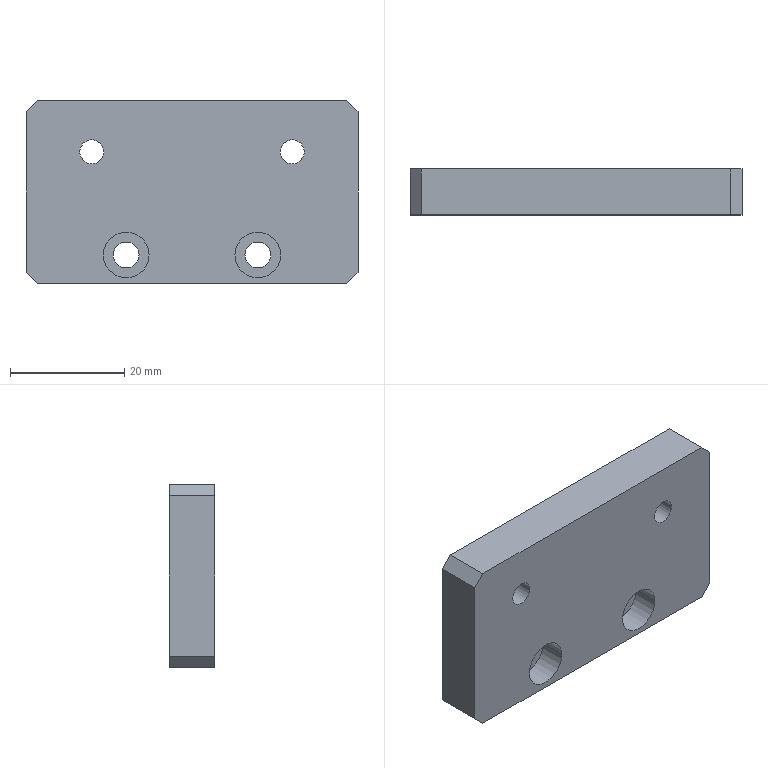Component | SolidWorks | 2018SOLIDWORKS1400000024-1 | 1 solid | 24 faces | box 58 x 8 x 32 mm | volume 13992 mm3 | cylinder 12 | plane 12 | commonest cylinder face diameters 4.2 x4 8 x4 4.5 x4 | material 6061 Alloy
build123d program:
from build123d import *

# Parameters (mm, degrees)
SKETCH1_W                                         = 58
SKETCH1_H                                         = 32
BOSS_EXTRUDE1_DEPTH                               = 4
HOLE_SIZE_ACCORDING_TO_TYPE_1_HEXAGON_D           = 4.5
HOLE_SIZE_ACCORDING_TO_TYPE_1_HEXAGON_CBORE_D     = 8
HOLE_SIZE_ACCORDING_TO_TYPE_1_HEXAGON_CBORE_DEPTH = 4.6
M5_TAPPED_HOLE1_D                                 = 4.2
CHAMFER1_SIZE                                     = 2


with BuildPart() as part:
    # Sketch1 → Boss-Extrude1 (new, symmetric)
    with BuildSketch(Plane.XY):
        Rectangle(SKETCH1_W, SKETCH1_H)
    extrude(amount=BOSS_EXTRUDE1_DEPTH, both=True)

    # Hole Size _ according to_ Type 1 Hexagon (through all)
    with Locations(Plane.XY.offset(4)):
        with Locations((-11.5, -11), (11.5, -11)):
            CounterBoreHole(HOLE_SIZE_ACCORDING_TO_TYPE_1_HEXAGON_D / 2, HOLE_SIZE_ACCORDING_TO_TYPE_1_HEXAGON_CBORE_D / 2, HOLE_SIZE_ACCORDING_TO_TYPE_1_HEXAGON_CBORE_DEPTH)

    # M5 Tapped Hole1 (through all)
    with Locations(Plane.XY.offset(4)):
        with Locations((-17.5, 7), (17.5, 7)):
            Hole(M5_TAPPED_HOLE1_D / 2)

    # Chamfer1
    chamfer1_edges = [part.edges().sort_by_distance(p)[0] for p in [
        (29, -16, 0),
        (-29, -16, 0),
        (-29, 16, 0),
        (29, 16, 0),
    ]]
    chamfer(chamfer1_edges, length=CHAMFER1_SIZE)


solid = part.part

# Placed as in the assembly
solid = solid.moved(Location((163.212, -80.5, 190), (90, 0, 0)))
STEP:
#1=COLOUR_RGB('',0.7922,0.8196,0.9333);
#2=FILL_AREA_STYLE_COLOUR('',#1);
#3=FILL_AREA_STYLE('',(#2));
#4=SURFACE_STYLE_FILL_AREA(#3);
#5=SURFACE_SIDE_STYLE('',(#4));
#6=SURFACE_STYLE_USAGE(.BOTH.,#5);
#7=PRESENTATION_STYLE_ASSIGNMENT((#6));
#8=CARTESIAN_POINT('',(5.654,-3.012,7.756));
#9=VERTEX_POINT('',#8);
#10=CARTESIAN_POINT('',(5.819,-3.012,7.756));
#11=VERTEX_POINT('',#10);
#12=CARTESIAN_POINT('',(5.737,-3.012,7.756));
#13=DIRECTION('',(0.,-1.,0.));
#14=DIRECTION('',(1.,0.,0.));
#15=AXIS2_PLACEMENT_3D('',#12,#13,#14);
#16=CIRCLE('',#15,0.08268);
#17=EDGE_CURVE('',#9,#11,#16,.T.);
#18=ORIENTED_EDGE('',*,*,#17,.F.);
#19=CARTESIAN_POINT('',(5.654,-3.327,7.756));
#20=VERTEX_POINT('',#19);
#21=CARTESIAN_POINT('',(5.654,-3.327,7.756));
#22=DIRECTION('',(0.,-1.,0.));
#23=VECTOR('',#22,39.37);
#24=LINE('',#21,#23);
#25=EDGE_CURVE('',#9,#20,#24,.T.);
#26=ORIENTED_EDGE('',*,*,#25,.T.);
#27=CARTESIAN_POINT('',(5.819,-3.327,7.756));
#28=VERTEX_POINT('',#27);
#29=CARTESIAN_POINT('',(5.737,-3.327,7.756));
#30=DIRECTION('',(0.,-1.,0.));
#31=DIRECTION('',(1.,0.,0.));
#32=AXIS2_PLACEMENT_3D('',#29,#30,#31);
#33=CIRCLE('',#32,0.08268);
#34=EDGE_CURVE('',#20,#28,#33,.T.);
#35=ORIENTED_EDGE('',*,*,#34,.T.);
#36=CARTESIAN_POINT('',(5.819,-3.327,7.756));
#37=DIRECTION('',(0.,-1.,0.));
#38=VECTOR('',#37,39.37);
#39=LINE('',#36,#38);
#40=EDGE_CURVE('',#11,#28,#39,.T.);
#41=ORIENTED_EDGE('',*,*,#40,.F.);
#42=EDGE_LOOP('',(#18,#26,#35,#41));
#43=FACE_OUTER_BOUND('',#42,.T.);
#44=CARTESIAN_POINT('',(5.737,-3.327,7.756));
#45=DIRECTION('',(0.,-1.,0.));
#46=DIRECTION('',(1.,0.,0.));
#47=AXIS2_PLACEMENT_3D('',#44,#45,#46);
#48=CYLINDRICAL_SURFACE('',#47,0.08268);
#49=ADVANCED_FACE('',(#43),#48,.F.);
#50=CARTESIAN_POINT('',(7.032,-3.012,7.756));
#51=VERTEX_POINT('',#50);
#52=CARTESIAN_POINT('',(7.197,-3.012,7.756));
#53=VERTEX_POINT('',#52);
#54=CARTESIAN_POINT('',(7.115,-3.012,7.756));
#55=DIRECTION('',(0.,-1.,0.));
#56=DIRECTION('',(1.,0.,0.));
#57=AXIS2_PLACEMENT_3D('',#54,#55,#56);
#58=CIRCLE('',#57,0.08268);
#59=EDGE_CURVE('',#51,#53,#58,.T.);
#60=ORIENTED_EDGE('',*,*,#59,.F.);
#61=CARTESIAN_POINT('',(7.032,-3.327,7.756));
#62=VERTEX_POINT('',#61);
#63=CARTESIAN_POINT('',(7.032,-3.327,7.756));
#64=DIRECTION('',(0.,-1.,0.));
#65=VECTOR('',#64,39.37);
#66=LINE('',#63,#65);
#67=EDGE_CURVE('',#51,#62,#66,.T.);
#68=ORIENTED_EDGE('',*,*,#67,.T.);
#69=CARTESIAN_POINT('',(7.197,-3.327,7.756));
#70=VERTEX_POINT('',#69);
#71=CARTESIAN_POINT('',(7.115,-3.327,7.756));
#72=DIRECTION('',(0.,-1.,0.));
#73=DIRECTION('',(1.,0.,0.));
#74=AXIS2_PLACEMENT_3D('',#71,#72,#73);
#75=CIRCLE('',#74,0.08268);
#76=EDGE_CURVE('',#62,#70,#75,.T.);
#77=ORIENTED_EDGE('',*,*,#76,.T.);
#78=CARTESIAN_POINT('',(7.197,-3.327,7.756));
#79=DIRECTION('',(0.,-1.,0.));
#80=VECTOR('',#79,39.37);
#81=LINE('',#78,#80);
#82=EDGE_CURVE('',#53,#70,#81,.T.);
#83=ORIENTED_EDGE('',*,*,#82,.F.);
#84=EDGE_LOOP('',(#60,#68,#77,#83));
#85=FACE_OUTER_BOUND('',#84,.T.);
#86=CARTESIAN_POINT('',(7.115,-3.327,7.756));
#87=DIRECTION('',(0.,-1.,0.));
#88=DIRECTION('',(1.,0.,0.));
#89=AXIS2_PLACEMENT_3D('',#86,#87,#88);
#90=CYLINDRICAL_SURFACE('',#89,0.08268);
#91=ADVANCED_FACE('',(#85),#90,.F.);
#92=CARTESIAN_POINT('',(5.815,-3.146,7.047));
#93=VERTEX_POINT('',#92);
#94=CARTESIAN_POINT('',(6.13,-3.146,7.047));
#95=VERTEX_POINT('',#94);
#96=CARTESIAN_POINT('',(5.973,-3.146,7.047));
#97=DIRECTION('',(0.,-1.,0.));
#98=DIRECTION('',(1.,0.,0.));
#99=AXIS2_PLACEMENT_3D('',#96,#97,#98);
#100=CIRCLE('',#99,0.1575);
#101=EDGE_CURVE('',#93,#95,#100,.T.);
#102=ORIENTED_EDGE('',*,*,#101,.F.);
#103=CARTESIAN_POINT('',(5.815,-3.327,7.047));
#104=VERTEX_POINT('',#103);
#105=CARTESIAN_POINT('',(5.815,-3.327,7.047));
#106=DIRECTION('',(0.,-1.,0.));
#107=VECTOR('',#106,39.37);
#108=LINE('',#105,#107);
#109=EDGE_CURVE('',#93,#104,#108,.T.);
#110=ORIENTED_EDGE('',*,*,#109,.T.);
#111=CARTESIAN_POINT('',(6.13,-3.327,7.047));
#112=VERTEX_POINT('',#111);
#113=CARTESIAN_POINT('',(5.973,-3.327,7.047));
#114=DIRECTION('',(0.,-1.,0.));
#115=DIRECTION('',(1.,0.,0.));
#116=AXIS2_PLACEMENT_3D('',#113,#114,#115);
#117=CIRCLE('',#116,0.1575);
#118=EDGE_CURVE('',#104,#112,#117,.T.);
#119=ORIENTED_EDGE('',*,*,#118,.T.);
#120=CARTESIAN_POINT('',(6.13,-3.327,7.047));
#121=DIRECTION('',(0.,-1.,0.));
#122=VECTOR('',#121,39.37);
#123=LINE('',#120,#122);
#124=EDGE_CURVE('',#95,#112,#123,.T.);
#125=ORIENTED_EDGE('',*,*,#124,.F.);
#126=EDGE_LOOP('',(#102,#110,#119,#125));
#127=FACE_OUTER_BOUND('',#126,.T.);
#128=CARTESIAN_POINT('',(5.973,-3.327,7.047));
#129=DIRECTION('',(0.,-1.,0.));
#130=DIRECTION('',(1.,0.,0.));
#131=AXIS2_PLACEMENT_3D('',#128,#129,#130);
#132=CYLINDRICAL_SURFACE('',#131,0.1575);
#133=ADVANCED_FACE('',(#127),#132,.F.);
#134=CARTESIAN_POINT('',(5.884,-3.012,7.047));
#135=VERTEX_POINT('',#134);
#136=CARTESIAN_POINT('',(6.061,-3.012,7.047));
#137=VERTEX_POINT('',#136);
#138=CARTESIAN_POINT('',(5.973,-3.012,7.047));
#139=DIRECTION('',(0.,-1.,0.));
#140=DIRECTION('',(1.,0.,0.));
#141=AXIS2_PLACEMENT_3D('',#138,#139,#140);
#142=CIRCLE('',#141,0.08858);
#143=EDGE_CURVE('',#135,#137,#142,.T.);
#144=ORIENTED_EDGE('',*,*,#143,.F.);
#145=CARTESIAN_POINT('',(5.884,-3.146,7.047));
#146=VERTEX_POINT('',#145);
#147=CARTESIAN_POINT('',(5.884,-3.327,7.047));
#148=DIRECTION('',(0.,-1.,0.));
#149=VECTOR('',#148,39.37);
#150=LINE('',#147,#149);
#151=EDGE_CURVE('',#135,#146,#150,.T.);
#152=ORIENTED_EDGE('',*,*,#151,.T.);
#153=CARTESIAN_POINT('',(6.061,-3.146,7.047));
#154=VERTEX_POINT('',#153);
#155=CARTESIAN_POINT('',(5.973,-3.146,7.047));
#156=DIRECTION('',(0.,-1.,0.));
#157=DIRECTION('',(1.,0.,0.));
#158=AXIS2_PLACEMENT_3D('',#155,#156,#157);
#159=CIRCLE('',#158,0.08858);
#160=EDGE_CURVE('',#146,#154,#159,.T.);
#161=ORIENTED_EDGE('',*,*,#160,.T.);
#162=CARTESIAN_POINT('',(6.061,-3.327,7.047));
#163=DIRECTION('',(0.,-1.,0.));
#164=VECTOR('',#163,39.37);
#165=LINE('',#162,#164);
#166=EDGE_CURVE('',#137,#154,#165,.T.);
#167=ORIENTED_EDGE('',*,*,#166,.F.);
#168=EDGE_LOOP('',(#144,#152,#161,#167));
#169=FACE_OUTER_BOUND('',#168,.T.);
#170=CARTESIAN_POINT('',(5.973,-3.327,7.047));
#171=DIRECTION('',(0.,-1.,0.));
#172=DIRECTION('',(1.,0.,0.));
#173=AXIS2_PLACEMENT_3D('',#170,#171,#172);
#174=CYLINDRICAL_SURFACE('',#173,0.08858);
#175=ADVANCED_FACE('',(#169),#174,.F.);
#176=CARTESIAN_POINT('',(6.721,-3.146,7.047));
#177=VERTEX_POINT('',#176);
#178=CARTESIAN_POINT('',(7.036,-3.146,7.047));
#179=VERTEX_POINT('',#178);
#180=CARTESIAN_POINT('',(6.878,-3.146,7.047));
#181=DIRECTION('',(0.,-1.,0.));
#182=DIRECTION('',(1.,0.,0.));
#183=AXIS2_PLACEMENT_3D('',#180,#181,#182);
#184=CIRCLE('',#183,0.1575);
#185=EDGE_CURVE('',#177,#179,#184,.T.);
#186=ORIENTED_EDGE('',*,*,#185,.F.);
#187=CARTESIAN_POINT('',(6.721,-3.327,7.047));
#188=VERTEX_POINT('',#187);
#189=CARTESIAN_POINT('',(6.721,-3.327,7.047));
#190=DIRECTION('',(0.,-1.,0.));
#191=VECTOR('',#190,39.37);
#192=LINE('',#189,#191);
#193=EDGE_CURVE('',#177,#188,#192,.T.);
#194=ORIENTED_EDGE('',*,*,#193,.T.);
#195=CARTESIAN_POINT('',(7.036,-3.327,7.047));
#196=VERTEX_POINT('',#195);
#197=CARTESIAN_POINT('',(6.878,-3.327,7.047));
#198=DIRECTION('',(0.,-1.,0.));
#199=DIRECTION('',(1.,0.,0.));
#200=AXIS2_PLACEMENT_3D('',#197,#198,#199);
#201=CIRCLE('',#200,0.1575);
#202=EDGE_CURVE('',#188,#196,#201,.T.);
#203=ORIENTED_EDGE('',*,*,#202,.T.);
#204=CARTESIAN_POINT('',(7.036,-3.327,7.047));
#205=DIRECTION('',(0.,-1.,0.));
#206=VECTOR('',#205,39.37);
#207=LINE('',#204,#206);
#208=EDGE_CURVE('',#179,#196,#207,.T.);
#209=ORIENTED_EDGE('',*,*,#208,.F.);
#210=EDGE_LOOP('',(#186,#194,#203,#209));
#211=FACE_OUTER_BOUND('',#210,.T.);
#212=CARTESIAN_POINT('',(6.878,-3.327,7.047));
#213=DIRECTION('',(0.,-1.,0.));
#214=DIRECTION('',(1.,0.,0.));
#215=AXIS2_PLACEMENT_3D('',#212,#213,#214);
#216=CYLINDRICAL_SURFACE('',#215,0.1575);
#217=ADVANCED_FACE('',(#211),#216,.F.);
#218=CARTESIAN_POINT('',(6.79,-3.012,7.047));
#219=VERTEX_POINT('',#218);
#220=CARTESIAN_POINT('',(6.967,-3.012,7.047));
#221=VERTEX_POINT('',#220);
#222=CARTESIAN_POINT('',(6.878,-3.012,7.047));
#223=DIRECTION('',(0.,-1.,0.));
#224=DIRECTION('',(1.,0.,0.));
#225=AXIS2_PLACEMENT_3D('',#222,#223,#224);
#226=CIRCLE('',#225,0.08858);
#227=EDGE_CURVE('',#219,#221,#226,.T.);
#228=ORIENTED_EDGE('',*,*,#227,.F.);
#229=CARTESIAN_POINT('',(6.79,-3.146,7.047));
#230=VERTEX_POINT('',#229);
#231=CARTESIAN_POINT('',(6.79,-3.327,7.047));
#232=DIRECTION('',(0.,-1.,0.));
#233=VECTOR('',#232,39.37);
#234=LINE('',#231,#233);
#235=EDGE_CURVE('',#219,#230,#234,.T.);
#236=ORIENTED_EDGE('',*,*,#235,.T.);
#237=CARTESIAN_POINT('',(6.967,-3.146,7.047));
#238=VERTEX_POINT('',#237);
#239=CARTESIAN_POINT('',(6.878,-3.146,7.047));
#240=DIRECTION('',(0.,-1.,0.));
#241=DIRECTION('',(1.,0.,0.));
#242=AXIS2_PLACEMENT_3D('',#239,#240,#241);
#243=CIRCLE('',#242,0.08858);
#244=EDGE_CURVE('',#230,#238,#243,.T.);
#245=ORIENTED_EDGE('',*,*,#244,.T.);
#246=CARTESIAN_POINT('',(6.967,-3.327,7.047));
#247=DIRECTION('',(0.,-1.,0.));
#248=VECTOR('',#247,39.37);
#249=LINE('',#246,#248);
#250=EDGE_CURVE('',#221,#238,#249,.T.);
#251=ORIENTED_EDGE('',*,*,#250,.F.);
#252=EDGE_LOOP('',(#228,#236,#245,#251));
#253=FACE_OUTER_BOUND('',#252,.T.);
#254=CARTESIAN_POINT('',(6.878,-3.327,7.047));
#255=DIRECTION('',(0.,-1.,0.));
#256=DIRECTION('',(1.,0.,0.));
#257=AXIS2_PLACEMENT_3D('',#254,#255,#256);
#258=CYLINDRICAL_SURFACE('',#257,0.08858);
#259=ADVANCED_FACE('',(#253),#258,.F.);
#260=CARTESIAN_POINT('',(7.567,-3.327,6.929));
#261=VERTEX_POINT('',#260);
#262=CARTESIAN_POINT('',(7.567,-3.327,8.031));
#263=VERTEX_POINT('',#262);
#264=CARTESIAN_POINT('',(7.567,-3.327,8.11));
#265=DIRECTION('',(-0.,0.,1.));
#266=VECTOR('',#265,39.37);
#267=LINE('',#264,#266);
#268=EDGE_CURVE('',#261,#263,#267,.T.);
#269=ORIENTED_EDGE('',*,*,#268,.F.);
#270=CARTESIAN_POINT('',(7.567,-3.012,6.929));
#271=VERTEX_POINT('',#270);
#272=CARTESIAN_POINT('',(7.567,-3.327,6.929));
#273=DIRECTION('',(-0.,1.,0.));
#274=VECTOR('',#273,39.37);
#275=LINE('',#272,#274);
#276=EDGE_CURVE('',#261,#271,#275,.T.);
#277=ORIENTED_EDGE('',*,*,#276,.T.);
#278=CARTESIAN_POINT('',(7.567,-3.012,8.031));
#279=VERTEX_POINT('',#278);
#280=CARTESIAN_POINT('',(7.567,-3.012,8.11));
#281=DIRECTION('',(-0.,0.,1.));
#282=VECTOR('',#281,39.37);
#283=LINE('',#280,#282);
#284=EDGE_CURVE('',#271,#279,#283,.T.);
#285=ORIENTED_EDGE('',*,*,#284,.T.);
#286=CARTESIAN_POINT('',(7.567,-3.327,8.031));
#287=DIRECTION('',(0.,-1.,0.));
#288=VECTOR('',#287,39.37);
#289=LINE('',#286,#288);
#290=EDGE_CURVE('',#279,#263,#289,.T.);
#291=ORIENTED_EDGE('',*,*,#290,.T.);
#292=EDGE_LOOP('',(#269,#277,#285,#291));
#293=FACE_OUTER_BOUND('',#292,.T.);
#294=CARTESIAN_POINT('',(7.567,-3.327,8.11));
#295=DIRECTION('',(-1.,-0.,-0.));
#296=DIRECTION('',(0.,-0.,-1.));
#297=AXIS2_PLACEMENT_3D('',#294,#295,#296);
#298=PLANE('',#297);
#299=ADVANCED_FACE('',(#293),#298,.F.);
#300=CARTESIAN_POINT('',(7.489,-3.327,8.11));
#301=VERTEX_POINT('',#300);
#302=CARTESIAN_POINT('',(5.363,-3.327,8.11));
#303=VERTEX_POINT('',#302);
#304=CARTESIAN_POINT('',(5.284,-3.327,8.11));
#305=DIRECTION('',(-1.,-0.,0.));
#306=VECTOR('',#305,39.37);
#307=LINE('',#304,#306);
#308=EDGE_CURVE('',#301,#303,#307,.T.);
#309=ORIENTED_EDGE('',*,*,#308,.F.);
#310=CARTESIAN_POINT('',(7.489,-3.012,8.11));
#311=VERTEX_POINT('',#310);
#312=CARTESIAN_POINT('',(7.489,-3.327,8.11));
#313=DIRECTION('',(-0.,1.,0.));
#314=VECTOR('',#313,39.37);
#315=LINE('',#312,#314);
#316=EDGE_CURVE('',#301,#311,#315,.T.);
#317=ORIENTED_EDGE('',*,*,#316,.T.);
#318=CARTESIAN_POINT('',(5.363,-3.012,8.11));
#319=VERTEX_POINT('',#318);
#320=CARTESIAN_POINT('',(5.284,-3.012,8.11));
#321=DIRECTION('',(-1.,-0.,0.));
#322=VECTOR('',#321,39.37);
#323=LINE('',#320,#322);
#324=EDGE_CURVE('',#311,#319,#323,.T.);
#325=ORIENTED_EDGE('',*,*,#324,.T.);
#326=CARTESIAN_POINT('',(5.363,-3.327,8.11));
#327=DIRECTION('',(0.,-1.,0.));
#328=VECTOR('',#327,39.37);
#329=LINE('',#326,#328);
#330=EDGE_CURVE('',#319,#303,#329,.T.);
#331=ORIENTED_EDGE('',*,*,#330,.T.);
#332=EDGE_LOOP('',(#309,#317,#325,#331));
#333=FACE_OUTER_BOUND('',#332,.T.);
#334=CARTESIAN_POINT('',(5.284,-3.327,8.11));
#335=DIRECTION('',(0.,0.,-1.));
#336=DIRECTION('',(-0.,1.,0.));
#337=AXIS2_PLACEMENT_3D('',#334,#335,#336);
#338=PLANE('',#337);
#339=ADVANCED_FACE('',(#333),#338,.F.);
#340=CARTESIAN_POINT('',(5.284,-3.012,8.031));
#341=VERTEX_POINT('',#340);
#342=CARTESIAN_POINT('',(5.284,-3.012,6.929));
#343=VERTEX_POINT('',#342);
#344=CARTESIAN_POINT('',(5.284,-3.012,8.11));
#345=DIRECTION('',(0.,-0.,-1.));
#346=VECTOR('',#345,39.37);
#347=LINE('',#344,#346);
#348=EDGE_CURVE('',#341,#343,#347,.T.);
#349=ORIENTED_EDGE('',*,*,#348,.T.);
#350=CARTESIAN_POINT('',(5.284,-3.327,6.929));
#351=VERTEX_POINT('',#350);
#352=CARTESIAN_POINT('',(5.284,-3.327,6.929));
#353=DIRECTION('',(0.,-1.,0.));
#354=VECTOR('',#353,39.37);
#355=LINE('',#352,#354);
#356=EDGE_CURVE('',#343,#351,#355,.T.);
#357=ORIENTED_EDGE('',*,*,#356,.T.);
#358=CARTESIAN_POINT('',(5.284,-3.327,8.031));
#359=VERTEX_POINT('',#358);
#360=CARTESIAN_POINT('',(5.284,-3.327,8.11));
#361=DIRECTION('',(0.,-0.,-1.));
#362=VECTOR('',#361,39.37);
#363=LINE('',#360,#362);
#364=EDGE_CURVE('',#359,#351,#363,.T.);
#365=ORIENTED_EDGE('',*,*,#364,.F.);
#366=CARTESIAN_POINT('',(5.284,-3.327,8.031));
#367=DIRECTION('',(-0.,1.,0.));
#368=VECTOR('',#367,39.37);
#369=LINE('',#366,#368);
#370=EDGE_CURVE('',#359,#341,#369,.T.);
#371=ORIENTED_EDGE('',*,*,#370,.T.);
#372=EDGE_LOOP('',(#349,#357,#365,#371));
#373=FACE_OUTER_BOUND('',#372,.T.);
#374=CARTESIAN_POINT('',(5.284,-3.327,8.11));
#375=DIRECTION('',(1.,0.,0.));
#376=DIRECTION('',(-0.,0.,1.));
#377=AXIS2_PLACEMENT_3D('',#374,#375,#376);
#378=PLANE('',#377);
#379=ADVANCED_FACE('',(#373),#378,.F.);
#380=CARTESIAN_POINT('',(5.363,-3.012,6.85));
#381=VERTEX_POINT('',#380);
#382=CARTESIAN_POINT('',(7.489,-3.012,6.85));
#383=VERTEX_POINT('',#382);
#384=CARTESIAN_POINT('',(5.284,-3.012,6.85));
#385=DIRECTION('',(1.,0.,-0.));
#386=VECTOR('',#385,39.37);
#387=LINE('',#384,#386);
#388=EDGE_CURVE('',#381,#383,#387,.T.);
#389=ORIENTED_EDGE('',*,*,#388,.T.);
#390=CARTESIAN_POINT('',(7.489,-3.327,6.85));
#391=VERTEX_POINT('',#390);
#392=CARTESIAN_POINT('',(7.489,-3.327,6.85));
#393=DIRECTION('',(0.,-1.,0.));
#394=VECTOR('',#393,39.37);
#395=LINE('',#392,#394);
#396=EDGE_CURVE('',#383,#391,#395,.T.);
#397=ORIENTED_EDGE('',*,*,#396,.T.);
#398=CARTESIAN_POINT('',(5.363,-3.327,6.85));
#399=VERTEX_POINT('',#398);
#400=CARTESIAN_POINT('',(5.284,-3.327,6.85));
#401=DIRECTION('',(1.,0.,-0.));
#402=VECTOR('',#401,39.37);
#403=LINE('',#400,#402);
#404=EDGE_CURVE('',#399,#391,#403,.T.);
#405=ORIENTED_EDGE('',*,*,#404,.F.);
#406=CARTESIAN_POINT('',(5.363,-3.327,6.85));
#407=DIRECTION('',(-0.,1.,0.));
#408=VECTOR('',#407,39.37);
#409=LINE('',#406,#408);
#410=EDGE_CURVE('',#399,#381,#409,.T.);
#411=ORIENTED_EDGE('',*,*,#410,.T.);
#412=EDGE_LOOP('',(#389,#397,#405,#411));
#413=FACE_OUTER_BOUND('',#412,.T.);
#414=CARTESIAN_POINT('',(5.284,-3.327,6.85));
#415=DIRECTION('',(-0.,-0.,1.));
#416=DIRECTION('',(0.,-1.,0.));
#417=AXIS2_PLACEMENT_3D('',#414,#415,#416);
#418=PLANE('',#417);
#419=ADVANCED_FACE('',(#413),#418,.F.);
#420=CARTESIAN_POINT('',(5.737,-3.327,7.756));
#421=DIRECTION('',(0.,-1.,0.));
#422=DIRECTION('',(1.,0.,0.));
#423=AXIS2_PLACEMENT_3D('',#420,#421,#422);
#424=CIRCLE('',#423,0.08268);
#425=EDGE_CURVE('',#28,#20,#424,.T.);
#426=ORIENTED_EDGE('',*,*,#425,.F.);
#427=ORIENTED_EDGE('',*,*,#34,.F.);
#428=EDGE_LOOP('',(#426,#427));
#429=FACE_BOUND('',#428,.T.);
#430=CARTESIAN_POINT('',(7.115,-3.327,7.756));
#431=DIRECTION('',(0.,-1.,0.));
#432=DIRECTION('',(1.,0.,0.));
#433=AXIS2_PLACEMENT_3D('',#430,#431,#432);
#434=CIRCLE('',#433,0.08268);
#435=EDGE_CURVE('',#70,#62,#434,.T.);
#436=ORIENTED_EDGE('',*,*,#435,.F.);
#437=ORIENTED_EDGE('',*,*,#76,.F.);
#438=EDGE_LOOP('',(#436,#437));
#439=FACE_BOUND('',#438,.T.);
#440=CARTESIAN_POINT('',(5.973,-3.327,7.047));
#441=DIRECTION('',(0.,-1.,0.));
#442=DIRECTION('',(1.,0.,0.));
#443=AXIS2_PLACEMENT_3D('',#440,#441,#442);
#444=CIRCLE('',#443,0.1575);
#445=EDGE_CURVE('',#112,#104,#444,.T.);
#446=ORIENTED_EDGE('',*,*,#445,.F.);
#447=ORIENTED_EDGE('',*,*,#118,.F.);
#448=EDGE_LOOP('',(#446,#447));
#449=FACE_BOUND('',#448,.T.);
#450=CARTESIAN_POINT('',(6.878,-3.327,7.047));
#451=DIRECTION('',(0.,-1.,0.));
#452=DIRECTION('',(1.,0.,0.));
#453=AXIS2_PLACEMENT_3D('',#450,#451,#452);
#454=CIRCLE('',#453,0.1575);
#455=EDGE_CURVE('',#196,#188,#454,.T.);
#456=ORIENTED_EDGE('',*,*,#455,.F.);
#457=ORIENTED_EDGE('',*,*,#202,.F.);
#458=EDGE_LOOP('',(#456,#457));
#459=FACE_BOUND('',#458,.T.);
#460=ORIENTED_EDGE('',*,*,#404,.T.);
#461=CARTESIAN_POINT('',(7.272,-3.327,6.634));
#462=DIRECTION('',(0.7071,0.,0.7071));
#463=VECTOR('',#462,39.37);
#464=LINE('',#461,#463);
#465=EDGE_CURVE('',#391,#261,#464,.T.);
#466=ORIENTED_EDGE('',*,*,#465,.T.);
#467=ORIENTED_EDGE('',*,*,#268,.T.);
#468=CARTESIAN_POINT('',(7.272,-3.327,8.327));
#469=DIRECTION('',(-0.7071,-0.,0.7071));
#470=VECTOR('',#469,39.37);
#471=LINE('',#468,#470);
#472=EDGE_CURVE('',#263,#301,#471,.T.);
#473=ORIENTED_EDGE('',*,*,#472,.T.);
#474=ORIENTED_EDGE('',*,*,#308,.T.);
#475=CARTESIAN_POINT('',(5.579,-3.327,8.327));
#476=DIRECTION('',(-0.7071,-0.,-0.7071));
#477=VECTOR('',#476,39.37);
#478=LINE('',#475,#477);
#479=EDGE_CURVE('',#303,#359,#478,.T.);
#480=ORIENTED_EDGE('',*,*,#479,.T.);
#481=ORIENTED_EDGE('',*,*,#364,.T.);
#482=CARTESIAN_POINT('',(5.579,-3.327,6.634));
#483=DIRECTION('',(0.7071,0.,-0.7071));
#484=VECTOR('',#483,39.37);
#485=LINE('',#482,#484);
#486=EDGE_CURVE('',#351,#399,#485,.T.);
#487=ORIENTED_EDGE('',*,*,#486,.T.);
#488=EDGE_LOOP('',(#460,#466,#467,#473,#474,#480,#481,#487));
#489=FACE_OUTER_BOUND('',#488,.T.);
#490=CARTESIAN_POINT('',(6.426,-3.327,7.48));
#491=DIRECTION('',(0.,-1.,-0.));
#492=DIRECTION('',(1.,0.,-0.));
#493=AXIS2_PLACEMENT_3D('',#490,#491,#492);
#494=PLANE('',#493);
#495=ADVANCED_FACE('',(#429,#439,#449,#459,#489),#494,.T.);
#496=CARTESIAN_POINT('',(5.737,-3.012,7.756));
#497=DIRECTION('',(0.,-1.,0.));
#498=DIRECTION('',(1.,0.,0.));
#499=AXIS2_PLACEMENT_3D('',#496,#497,#498);
#500=CIRCLE('',#499,0.08268);
#501=EDGE_CURVE('',#11,#9,#500,.T.);
#502=ORIENTED_EDGE('',*,*,#501,.T.);
#503=ORIENTED_EDGE('',*,*,#17,.T.);
#504=EDGE_LOOP('',(#502,#503));
#505=FACE_BOUND('',#504,.T.);
#506=CARTESIAN_POINT('',(7.115,-3.012,7.756));
#507=DIRECTION('',(0.,-1.,0.));
#508=DIRECTION('',(1.,0.,0.));
#509=AXIS2_PLACEMENT_3D('',#506,#507,#508);
#510=CIRCLE('',#509,0.08268);
#511=EDGE_CURVE('',#53,#51,#510,.T.);
#512=ORIENTED_EDGE('',*,*,#511,.T.);
#513=ORIENTED_EDGE('',*,*,#59,.T.);
#514=EDGE_LOOP('',(#512,#513));
#515=FACE_BOUND('',#514,.T.);
#516=CARTESIAN_POINT('',(5.973,-3.012,7.047));
#517=DIRECTION('',(0.,-1.,0.));
#518=DIRECTION('',(1.,0.,0.));
#519=AXIS2_PLACEMENT_3D('',#516,#517,#518);
#520=CIRCLE('',#519,0.08858);
#521=EDGE_CURVE('',#137,#135,#520,.T.);
#522=ORIENTED_EDGE('',*,*,#521,.T.);
#523=ORIENTED_EDGE('',*,*,#143,.T.);
#524=EDGE_LOOP('',(#522,#523));
#525=FACE_BOUND('',#524,.T.);
#526=CARTESIAN_POINT('',(6.878,-3.012,7.047));
#527=DIRECTION('',(0.,-1.,0.));
#528=DIRECTION('',(1.,0.,0.));
#529=AXIS2_PLACEMENT_3D('',#526,#527,#528);
#530=CIRCLE('',#529,0.08858);
#531=EDGE_CURVE('',#221,#219,#530,.T.);
#532=ORIENTED_EDGE('',*,*,#531,.T.);
#533=ORIENTED_EDGE('',*,*,#227,.T.);
#534=EDGE_LOOP('',(#532,#533));
#535=FACE_BOUND('',#534,.T.);
#536=ORIENTED_EDGE('',*,*,#284,.F.);
#537=CARTESIAN_POINT('',(7.567,-3.012,6.929));
#538=DIRECTION('',(-0.7071,-0.,-0.7071));
#539=VECTOR('',#538,39.37);
#540=LINE('',#537,#539);
#541=EDGE_CURVE('',#271,#383,#540,.T.);
#542=ORIENTED_EDGE('',*,*,#541,.T.);
#543=ORIENTED_EDGE('',*,*,#388,.F.);
#544=CARTESIAN_POINT('',(5.363,-3.012,6.85));
#545=DIRECTION('',(-0.7071,-0.,0.7071));
#546=VECTOR('',#545,39.37);
#547=LINE('',#544,#546);
#548=EDGE_CURVE('',#381,#343,#547,.T.);
#549=ORIENTED_EDGE('',*,*,#548,.T.);
#550=ORIENTED_EDGE('',*,*,#348,.F.);
#551=CARTESIAN_POINT('',(5.284,-3.012,8.031));
#552=DIRECTION('',(0.7071,0.,0.7071));
#553=VECTOR('',#552,39.37);
#554=LINE('',#551,#553);
#555=EDGE_CURVE('',#341,#319,#554,.T.);
#556=ORIENTED_EDGE('',*,*,#555,.T.);
#557=ORIENTED_EDGE('',*,*,#324,.F.);
#558=CARTESIAN_POINT('',(7.489,-3.012,8.11));
#559=DIRECTION('',(0.7071,0.,-0.7071));
#560=VECTOR('',#559,39.37);
#561=LINE('',#558,#560);
#562=EDGE_CURVE('',#311,#279,#561,.T.);
#563=ORIENTED_EDGE('',*,*,#562,.T.);
#564=EDGE_LOOP('',(#536,#542,#543,#549,#550,#556,#557,#563));
#565=FACE_OUTER_BOUND('',#564,.T.);
#566=CARTESIAN_POINT('',(6.426,-3.012,7.48));
#567=DIRECTION('',(0.,-1.,-0.));
#568=DIRECTION('',(1.,0.,-0.));
#569=AXIS2_PLACEMENT_3D('',#566,#567,#568);
#570=PLANE('',#569);
#571=ADVANCED_FACE('',(#505,#515,#525,#535,#565),#570,.F.);
#572=ORIENTED_EDGE('',*,*,#235,.F.);
#573=ORIENTED_EDGE('',*,*,#531,.F.);
#574=ORIENTED_EDGE('',*,*,#250,.T.);
#575=CARTESIAN_POINT('',(6.878,-3.146,7.047));
#576=DIRECTION('',(0.,-1.,0.));
#577=DIRECTION('',(1.,0.,0.));
#578=AXIS2_PLACEMENT_3D('',#575,#576,#577);
#579=CIRCLE('',#578,0.08858);
#580=EDGE_CURVE('',#238,#230,#579,.T.);
#581=ORIENTED_EDGE('',*,*,#580,.T.);
#582=EDGE_LOOP('',(#572,#573,#574,#581));
#583=FACE_OUTER_BOUND('',#582,.T.);
#584=CARTESIAN_POINT('',(6.878,-3.327,7.047));
#585=DIRECTION('',(0.,-1.,0.));
#586=DIRECTION('',(1.,0.,0.));
#587=AXIS2_PLACEMENT_3D('',#584,#585,#586);
#588=CYLINDRICAL_SURFACE('',#587,0.08858);
#589=ADVANCED_FACE('',(#583),#588,.F.);
#590=ORIENTED_EDGE('',*,*,#580,.F.);
#591=ORIENTED_EDGE('',*,*,#244,.F.);
#592=EDGE_LOOP('',(#590,#591));
#593=FACE_BOUND('',#592,.T.);
#594=CARTESIAN_POINT('',(6.878,-3.146,7.047));
#595=DIRECTION('',(0.,-1.,0.));
#596=DIRECTION('',(1.,0.,0.));
#597=AXIS2_PLACEMENT_3D('',#594,#595,#596);
#598=CIRCLE('',#597,0.1575);
#599=EDGE_CURVE('',#179,#177,#598,.T.);
#600=ORIENTED_EDGE('',*,*,#599,.T.);
#601=ORIENTED_EDGE('',*,*,#185,.T.);
#602=EDGE_LOOP('',(#600,#601));
#603=FACE_OUTER_BOUND('',#602,.T.);
#604=CARTESIAN_POINT('',(6.967,-3.146,7.047));
#605=DIRECTION('',(-0.,1.,0.));
#606=DIRECTION('',(-1.,-0.,0.));
#607=AXIS2_PLACEMENT_3D('',#604,#605,#606);
#608=PLANE('',#607);
#609=ADVANCED_FACE('',(#593,#603),#608,.F.);
#610=ORIENTED_EDGE('',*,*,#193,.F.);
#611=ORIENTED_EDGE('',*,*,#599,.F.);
#612=ORIENTED_EDGE('',*,*,#208,.T.);
#613=ORIENTED_EDGE('',*,*,#455,.T.);
#614=EDGE_LOOP('',(#610,#611,#612,#613));
#615=FACE_OUTER_BOUND('',#614,.T.);
#616=CARTESIAN_POINT('',(6.878,-3.327,7.047));
#617=DIRECTION('',(0.,-1.,0.));
#618=DIRECTION('',(1.,0.,0.));
#619=AXIS2_PLACEMENT_3D('',#616,#617,#618);
#620=CYLINDRICAL_SURFACE('',#619,0.1575);
#621=ADVANCED_FACE('',(#615),#620,.F.);
#622=ORIENTED_EDGE('',*,*,#151,.F.);
#623=ORIENTED_EDGE('',*,*,#521,.F.);
#624=ORIENTED_EDGE('',*,*,#166,.T.);
#625=CARTESIAN_POINT('',(5.973,-3.146,7.047));
#626=DIRECTION('',(0.,-1.,0.));
#627=DIRECTION('',(1.,0.,0.));
#628=AXIS2_PLACEMENT_3D('',#625,#626,#627);
#629=CIRCLE('',#628,0.08858);
#630=EDGE_CURVE('',#154,#146,#629,.T.);
#631=ORIENTED_EDGE('',*,*,#630,.T.);
#632=EDGE_LOOP('',(#622,#623,#624,#631));
#633=FACE_OUTER_BOUND('',#632,.T.);
#634=CARTESIAN_POINT('',(5.973,-3.327,7.047));
#635=DIRECTION('',(0.,-1.,0.));
#636=DIRECTION('',(1.,0.,0.));
#637=AXIS2_PLACEMENT_3D('',#634,#635,#636);
#638=CYLINDRICAL_SURFACE('',#637,0.08858);
#639=ADVANCED_FACE('',(#633),#638,.F.);
#640=ORIENTED_EDGE('',*,*,#630,.F.);
#641=ORIENTED_EDGE('',*,*,#160,.F.);
#642=EDGE_LOOP('',(#640,#641));
#643=FACE_BOUND('',#642,.T.);
#644=CARTESIAN_POINT('',(5.973,-3.146,7.047));
#645=DIRECTION('',(0.,-1.,0.));
#646=DIRECTION('',(1.,0.,0.));
#647=AXIS2_PLACEMENT_3D('',#644,#645,#646);
#648=CIRCLE('',#647,0.1575);
#649=EDGE_CURVE('',#95,#93,#648,.T.);
#650=ORIENTED_EDGE('',*,*,#649,.T.);
#651=ORIENTED_EDGE('',*,*,#101,.T.);
#652=EDGE_LOOP('',(#650,#651));
#653=FACE_OUTER_BOUND('',#652,.T.);
#654=CARTESIAN_POINT('',(6.061,-3.146,7.047));
#655=DIRECTION('',(-0.,1.,0.));
#656=DIRECTION('',(-1.,-0.,0.));
#657=AXIS2_PLACEMENT_3D('',#654,#655,#656);
#658=PLANE('',#657);
#659=ADVANCED_FACE('',(#643,#653),#658,.F.);
#660=ORIENTED_EDGE('',*,*,#109,.F.);
#661=ORIENTED_EDGE('',*,*,#649,.F.);
#662=ORIENTED_EDGE('',*,*,#124,.T.);
#663=ORIENTED_EDGE('',*,*,#445,.T.);
#664=EDGE_LOOP('',(#660,#661,#662,#663));
#665=FACE_OUTER_BOUND('',#664,.T.);
#666=CARTESIAN_POINT('',(5.973,-3.327,7.047));
#667=DIRECTION('',(0.,-1.,0.));
#668=DIRECTION('',(1.,0.,0.));
#669=AXIS2_PLACEMENT_3D('',#666,#667,#668);
#670=CYLINDRICAL_SURFACE('',#669,0.1575);
#671=ADVANCED_FACE('',(#665),#670,.F.);
#672=ORIENTED_EDGE('',*,*,#67,.F.);
#673=ORIENTED_EDGE('',*,*,#511,.F.);
#674=ORIENTED_EDGE('',*,*,#82,.T.);
#675=ORIENTED_EDGE('',*,*,#435,.T.);
#676=EDGE_LOOP('',(#672,#673,#674,#675));
#677=FACE_OUTER_BOUND('',#676,.T.);
#678=CARTESIAN_POINT('',(7.115,-3.327,7.756));
#679=DIRECTION('',(0.,-1.,0.));
#680=DIRECTION('',(1.,0.,0.));
#681=AXIS2_PLACEMENT_3D('',#678,#679,#680);
#682=CYLINDRICAL_SURFACE('',#681,0.08268);
#683=ADVANCED_FACE('',(#677),#682,.F.);
#684=ORIENTED_EDGE('',*,*,#25,.F.);
#685=ORIENTED_EDGE('',*,*,#501,.F.);
#686=ORIENTED_EDGE('',*,*,#40,.T.);
#687=ORIENTED_EDGE('',*,*,#425,.T.);
#688=EDGE_LOOP('',(#684,#685,#686,#687));
#689=FACE_OUTER_BOUND('',#688,.T.);
#690=CARTESIAN_POINT('',(5.737,-3.327,7.756));
#691=DIRECTION('',(0.,-1.,0.));
#692=DIRECTION('',(1.,0.,0.));
#693=AXIS2_PLACEMENT_3D('',#690,#691,#692);
#694=CYLINDRICAL_SURFACE('',#693,0.08268);
#695=ADVANCED_FACE('',(#689),#694,.F.);
#696=ORIENTED_EDGE('',*,*,#465,.F.);
#697=ORIENTED_EDGE('',*,*,#396,.F.);
#698=ORIENTED_EDGE('',*,*,#541,.F.);
#699=ORIENTED_EDGE('',*,*,#276,.F.);
#700=EDGE_LOOP('',(#696,#697,#698,#699));
#701=FACE_OUTER_BOUND('',#700,.T.);
#702=CARTESIAN_POINT('',(7.567,-3.327,6.929));
#703=DIRECTION('',(-0.7071,-0.,0.7071));
#704=DIRECTION('',(-0.,1.,0.));
#705=AXIS2_PLACEMENT_3D('',#702,#703,#704);
#706=PLANE('',#705);
#707=ADVANCED_FACE('',(#701),#706,.F.);
#708=ORIENTED_EDGE('',*,*,#486,.F.);
#709=ORIENTED_EDGE('',*,*,#356,.F.);
#710=ORIENTED_EDGE('',*,*,#548,.F.);
#711=ORIENTED_EDGE('',*,*,#410,.F.);
#712=EDGE_LOOP('',(#708,#709,#710,#711));
#713=FACE_OUTER_BOUND('',#712,.T.);
#714=CARTESIAN_POINT('',(5.363,-3.327,6.85));
#715=DIRECTION('',(0.7071,0.,0.7071));
#716=DIRECTION('',(-0.,1.,0.));
#717=AXIS2_PLACEMENT_3D('',#714,#715,#716);
#718=PLANE('',#717);
#719=ADVANCED_FACE('',(#713),#718,.F.);
#720=ORIENTED_EDGE('',*,*,#472,.F.);
#721=ORIENTED_EDGE('',*,*,#290,.F.);
#722=ORIENTED_EDGE('',*,*,#562,.F.);
#723=ORIENTED_EDGE('',*,*,#316,.F.);
#724=EDGE_LOOP('',(#720,#721,#722,#723));
#725=FACE_OUTER_BOUND('',#724,.T.);
#726=CARTESIAN_POINT('',(7.489,-3.327,8.11));
#727=DIRECTION('',(-0.7071,-0.,-0.7071));
#728=DIRECTION('',(-0.,1.,0.));
#729=AXIS2_PLACEMENT_3D('',#726,#727,#728);
#730=PLANE('',#729);
#731=ADVANCED_FACE('',(#725),#730,.F.);
#732=ORIENTED_EDGE('',*,*,#479,.F.);
#733=ORIENTED_EDGE('',*,*,#330,.F.);
#734=ORIENTED_EDGE('',*,*,#555,.F.);
#735=ORIENTED_EDGE('',*,*,#370,.F.);
#736=EDGE_LOOP('',(#732,#733,#734,#735));
#737=FACE_OUTER_BOUND('',#736,.T.);
#738=CARTESIAN_POINT('',(5.284,-3.327,8.031));
#739=DIRECTION('',(0.7071,0.,-0.7071));
#740=DIRECTION('',(-0.,1.,0.));
#741=AXIS2_PLACEMENT_3D('',#738,#739,#740);
#742=PLANE('',#741);
#743=ADVANCED_FACE('',(#737),#742,.F.);
#744=CLOSED_SHELL('',(#49,#91,#133,#175,#217,#259,#299,#339,#379,#419,#495,#571,#589,#609,#621,#639,#659,#671,#683,#695,#707,#719,#731,#743));
#745=MANIFOLD_SOLID_BREP('',#744);
#746=STYLED_ITEM('',(#7),#745);
#747=PRESENTATION_LAYER_ASSIGNMENT('','',(#746));
#748=(LENGTH_UNIT()NAMED_UNIT(*)SI_UNIT($,.METRE.));
#749=LENGTH_MEASURE_WITH_UNIT(LENGTH_MEASURE(0.0254),#748);
#750=DIMENSIONAL_EXPONENTS(1.,0.,0.,0.,0.,0.,0.);
#751=(CONVERSION_BASED_UNIT('',#749)LENGTH_UNIT()NAMED_UNIT(#750));
#752=UNCERTAINTY_MEASURE_WITH_UNIT(LENGTH_MEASURE(0.00001),#751,'','');
#753=(NAMED_UNIT(*)PLANE_ANGLE_UNIT()SI_UNIT($,.RADIAN.));
#754=(NAMED_UNIT(*)SI_UNIT($,.STERADIAN.)SOLID_ANGLE_UNIT());
#755=(GEOMETRIC_REPRESENTATION_CONTEXT(3)GLOBAL_UNCERTAINTY_ASSIGNED_CONTEXT((#752))GLOBAL_UNIT_ASSIGNED_CONTEXT((#751,#753,#754))REPRESENTATION_CONTEXT('',''));
#756=MECHANICAL_DESIGN_GEOMETRIC_PRESENTATION_REPRESENTATION('',(#746),#755);
#757=CARTESIAN_POINT('',(0.,0.,0.));
#758=DIRECTION('',(0.,0.,1.));
#759=DIRECTION('',(1.,0.,0.));
#760=AXIS2_PLACEMENT_3D('',#757,#758,#759);
#761=(LENGTH_UNIT()NAMED_UNIT(*)SI_UNIT($,.METRE.));
#762=LENGTH_MEASURE_WITH_UNIT(LENGTH_MEASURE(0.0254),#761);
#763=DIMENSIONAL_EXPONENTS(1.,0.,0.,0.,0.,0.,0.);
#764=(CONVERSION_BASED_UNIT('',#762)LENGTH_UNIT()NAMED_UNIT(#763));
#765=UNCERTAINTY_MEASURE_WITH_UNIT(LENGTH_MEASURE(0.00001),#764,'','');
#766=(NAMED_UNIT(*)PLANE_ANGLE_UNIT()SI_UNIT($,.RADIAN.));
#767=(NAMED_UNIT(*)SI_UNIT($,.STERADIAN.)SOLID_ANGLE_UNIT());
#768=(GEOMETRIC_REPRESENTATION_CONTEXT(3)GLOBAL_UNCERTAINTY_ASSIGNED_CONTEXT((#765))GLOBAL_UNIT_ASSIGNED_CONTEXT((#764,#766,#767))REPRESENTATION_CONTEXT('',''));
#769=ADVANCED_BREP_SHAPE_REPRESENTATION('',(#745,#760),#768);